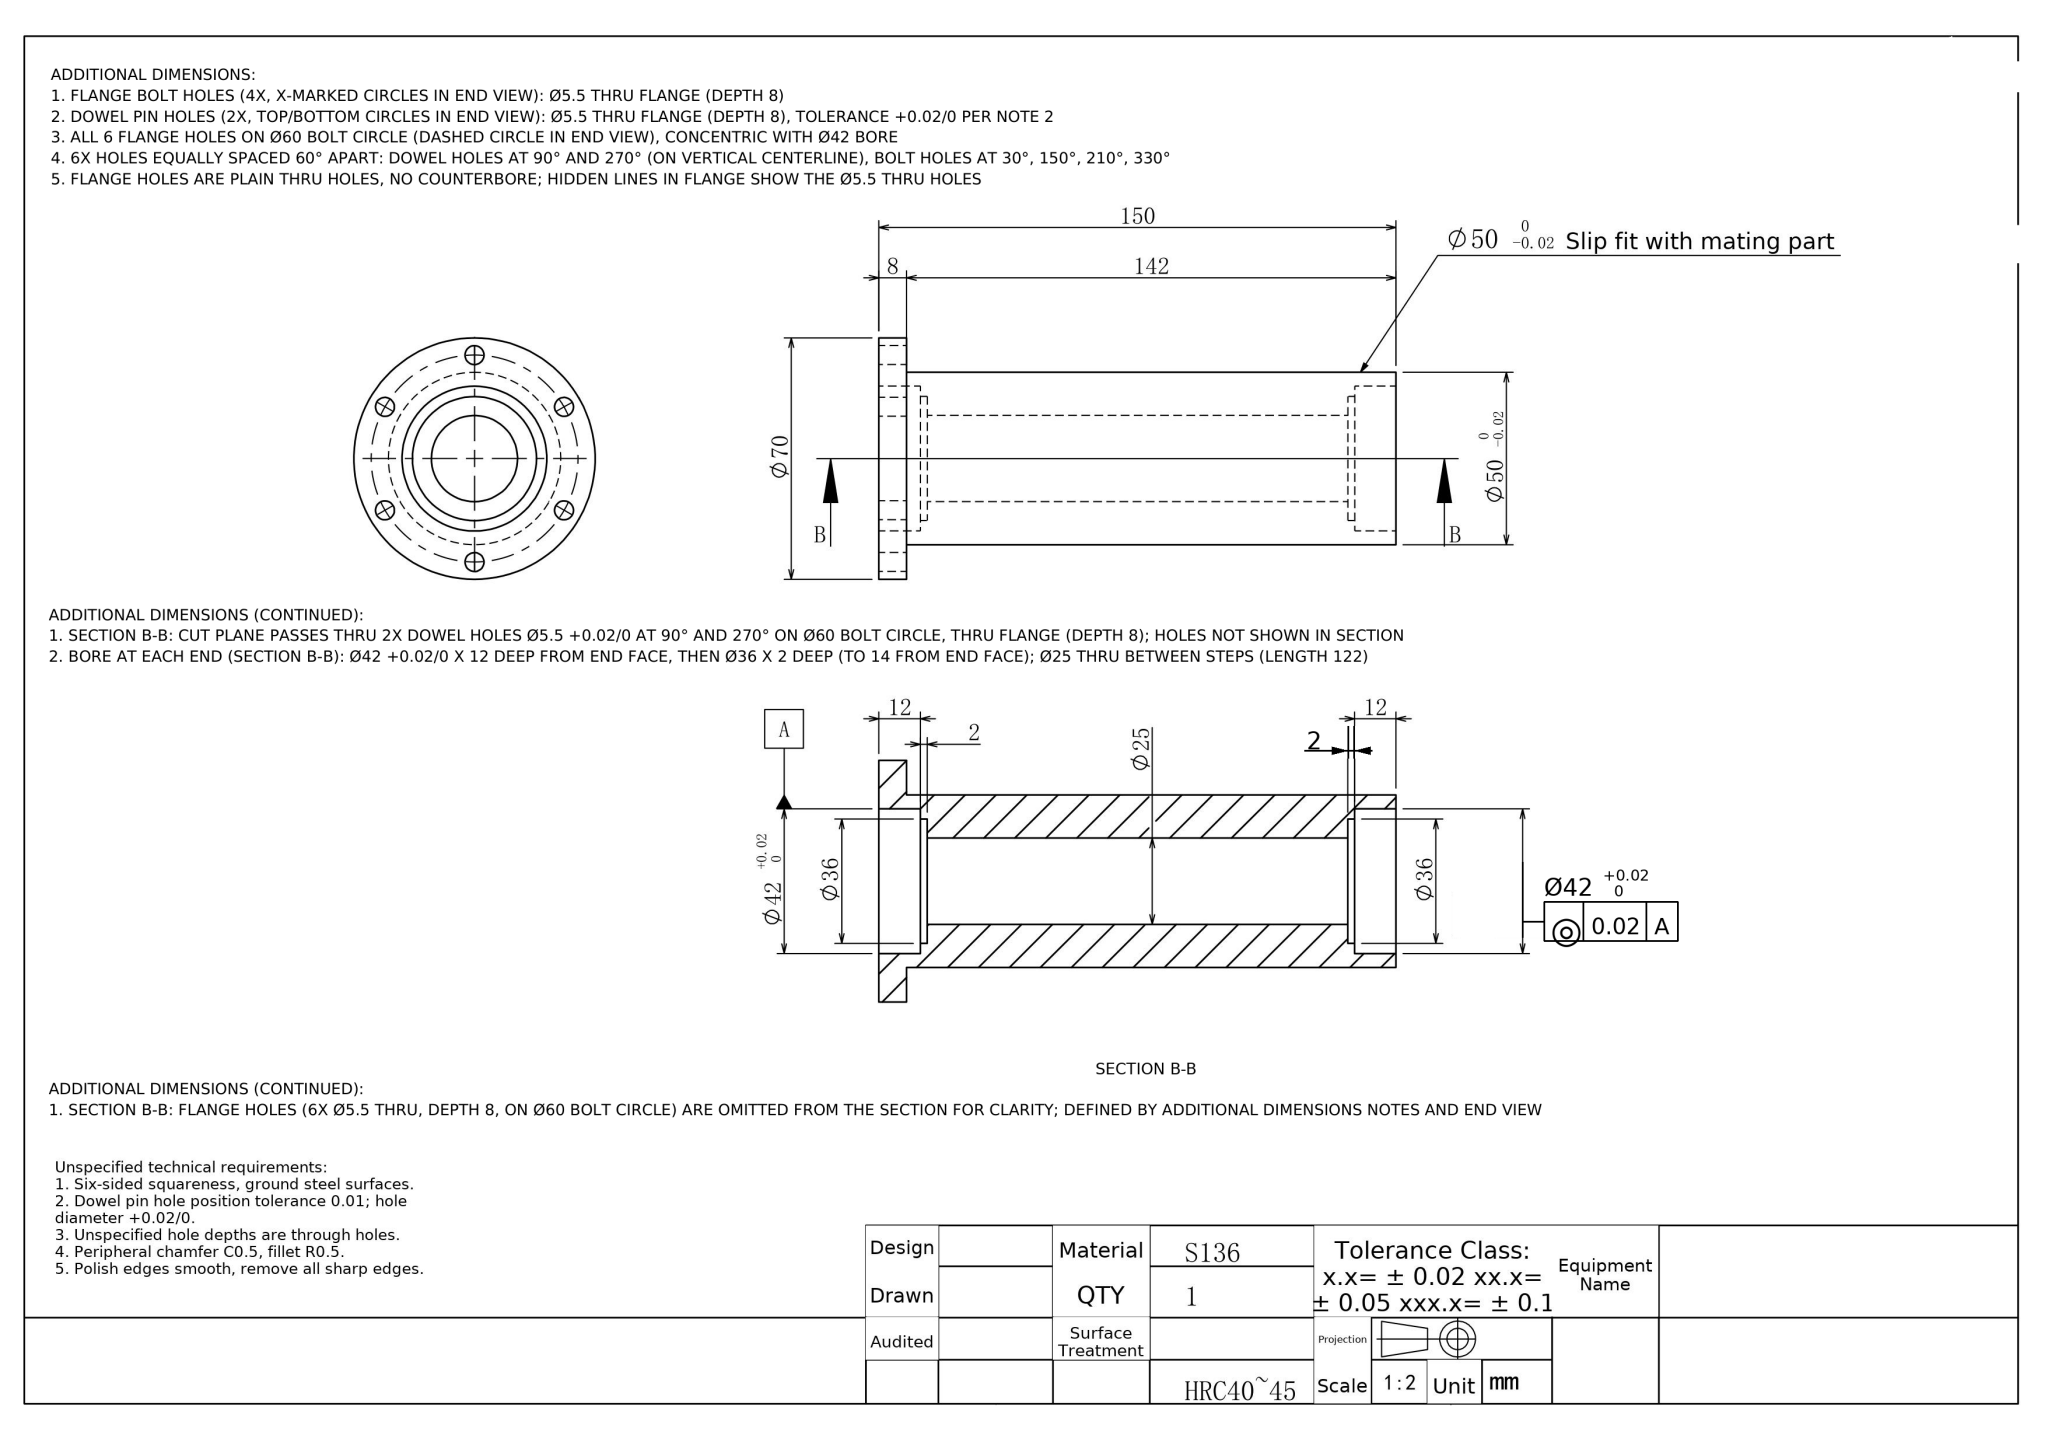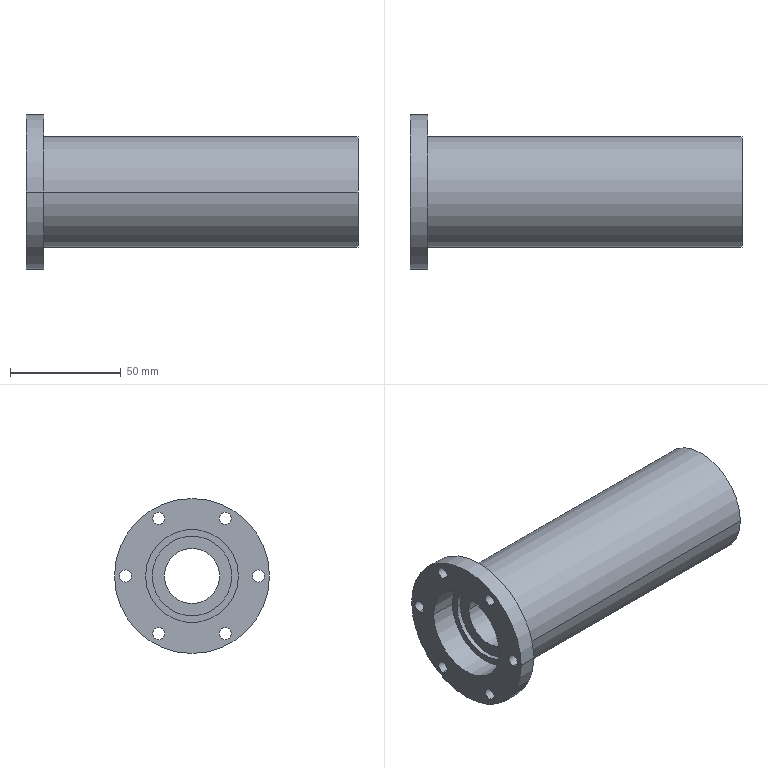Part | NX | mm | 1 solid | 33 faces | box 150 x 70 x 70 mm | volume 211255 mm3 | cylinder 26 | plane 7 | commonest cylinder face diameters 5.5 x12 36 x4 42 x4 50 x2 70 x2 25 x2
STEP:
#1=CARTESIAN_POINT('',(136.,-18.,0.));
#2=VERTEX_POINT('',#1);
#3=CARTESIAN_POINT('',(136.,18.,0.));
#4=VERTEX_POINT('',#3);
#5=CARTESIAN_POINT('',(136.,-0.,0.));
#6=DIRECTION('',(1.,-0.,0.));
#7=DIRECTION('',(0.,1.,0.));
#8=AXIS2_PLACEMENT_3D('',#5,#6,#7);
#9=CIRCLE('',#8,18.);
#10=EDGE_CURVE('',#2,#4,#9,.T.);
#11=ORIENTED_EDGE('',*,*,#10,.F.);
#12=CARTESIAN_POINT('',(138.,-18.,0.));
#13=VERTEX_POINT('',#12);
#14=CARTESIAN_POINT('',(136.,-18.,0.));
#15=DIRECTION('',(1.,-0.,0.));
#16=VECTOR('',#15,1000.);
#17=LINE('',#14,#16);
#18=EDGE_CURVE('',#2,#13,#17,.T.);
#19=ORIENTED_EDGE('',*,*,#18,.T.);
#20=CARTESIAN_POINT('',(138.,18.,0.));
#21=VERTEX_POINT('',#20);
#22=CARTESIAN_POINT('',(138.,-0.,0.));
#23=DIRECTION('',(1.,-0.,0.));
#24=DIRECTION('',(0.,1.,0.));
#25=AXIS2_PLACEMENT_3D('',#22,#23,#24);
#26=CIRCLE('',#25,18.);
#27=EDGE_CURVE('',#13,#21,#26,.T.);
#28=ORIENTED_EDGE('',*,*,#27,.T.);
#29=CARTESIAN_POINT('',(136.,18.,0.));
#30=DIRECTION('',(1.,-0.,0.));
#31=VECTOR('',#30,1000.);
#32=LINE('',#29,#31);
#33=EDGE_CURVE('',#4,#21,#32,.T.);
#34=ORIENTED_EDGE('',*,*,#33,.F.);
#35=EDGE_LOOP('',(#11,#19,#28,#34));
#36=FACE_OUTER_BOUND('',#35,.T.);
#37=CARTESIAN_POINT('',(136.,-0.,0.));
#38=DIRECTION('',(1.,-0.,0.));
#39=DIRECTION('',(0.,1.,0.));
#40=AXIS2_PLACEMENT_3D('',#37,#38,#39);
#41=CYLINDRICAL_SURFACE('',#40,18.);
#42=ADVANCED_FACE('',(#36),#41,.F.);
#43=CARTESIAN_POINT('',(14.,18.,0.));
#44=VERTEX_POINT('',#43);
#45=CARTESIAN_POINT('',(14.,-18.,0.));
#46=VERTEX_POINT('',#45);
#47=CARTESIAN_POINT('',(14.,-0.,0.));
#48=DIRECTION('',(-1.,0.,0.));
#49=DIRECTION('',(-0.,-1.,0.));
#50=AXIS2_PLACEMENT_3D('',#47,#48,#49);
#51=CIRCLE('',#50,18.);
#52=EDGE_CURVE('',#44,#46,#51,.T.);
#53=ORIENTED_EDGE('',*,*,#52,.F.);
#54=CARTESIAN_POINT('',(12.,18.,0.));
#55=VERTEX_POINT('',#54);
#56=CARTESIAN_POINT('',(14.,18.,0.));
#57=DIRECTION('',(-1.,0.,0.));
#58=VECTOR('',#57,1000.);
#59=LINE('',#56,#58);
#60=EDGE_CURVE('',#44,#55,#59,.T.);
#61=ORIENTED_EDGE('',*,*,#60,.T.);
#62=CARTESIAN_POINT('',(12.,-18.,0.));
#63=VERTEX_POINT('',#62);
#64=CARTESIAN_POINT('',(12.,-0.,0.));
#65=DIRECTION('',(-1.,0.,0.));
#66=DIRECTION('',(-0.,-1.,0.));
#67=AXIS2_PLACEMENT_3D('',#64,#65,#66);
#68=CIRCLE('',#67,18.);
#69=EDGE_CURVE('',#55,#63,#68,.T.);
#70=ORIENTED_EDGE('',*,*,#69,.T.);
#71=CARTESIAN_POINT('',(14.,-18.,0.));
#72=DIRECTION('',(-1.,0.,0.));
#73=VECTOR('',#72,1000.);
#74=LINE('',#71,#73);
#75=EDGE_CURVE('',#46,#63,#74,.T.);
#76=ORIENTED_EDGE('',*,*,#75,.F.);
#77=EDGE_LOOP('',(#53,#61,#70,#76));
#78=FACE_OUTER_BOUND('',#77,.T.);
#79=CARTESIAN_POINT('',(14.,-0.,0.));
#80=DIRECTION('',(-1.,0.,0.));
#81=DIRECTION('',(-0.,-1.,0.));
#82=AXIS2_PLACEMENT_3D('',#79,#80,#81);
#83=CYLINDRICAL_SURFACE('',#82,18.);
#84=ADVANCED_FACE('',(#78),#83,.F.);
#85=CARTESIAN_POINT('',(8.,15.,-23.231));
#86=VERTEX_POINT('',#85);
#87=CARTESIAN_POINT('',(8.,15.,-28.731));
#88=VERTEX_POINT('',#87);
#89=CARTESIAN_POINT('',(8.,15.,-25.981));
#90=DIRECTION('',(1.,-0.,0.));
#91=DIRECTION('',(0.,1.,0.));
#92=AXIS2_PLACEMENT_3D('',#89,#90,#91);
#93=CIRCLE('',#92,2.75);
#94=EDGE_CURVE('',#86,#88,#93,.T.);
#95=ORIENTED_EDGE('',*,*,#94,.T.);
#96=CARTESIAN_POINT('',(0.,15.,-28.731));
#97=VERTEX_POINT('',#96);
#98=CARTESIAN_POINT('',(0.,15.,-28.731));
#99=DIRECTION('',(-1.,0.,0.));
#100=VECTOR('',#99,1000.);
#101=LINE('',#98,#100);
#102=EDGE_CURVE('',#88,#97,#101,.T.);
#103=ORIENTED_EDGE('',*,*,#102,.T.);
#104=CARTESIAN_POINT('',(0.,15.,-23.231));
#105=VERTEX_POINT('',#104);
#106=CARTESIAN_POINT('',(0.,15.,-25.981));
#107=DIRECTION('',(-1.,0.,0.));
#108=DIRECTION('',(0.,0.,1.));
#109=AXIS2_PLACEMENT_3D('',#106,#107,#108);
#110=CIRCLE('',#109,2.75);
#111=EDGE_CURVE('',#97,#105,#110,.T.);
#112=ORIENTED_EDGE('',*,*,#111,.T.);
#113=CARTESIAN_POINT('',(0.,15.,-23.231));
#114=DIRECTION('',(-1.,0.,0.));
#115=VECTOR('',#114,1000.);
#116=LINE('',#113,#115);
#117=EDGE_CURVE('',#86,#105,#116,.T.);
#118=ORIENTED_EDGE('',*,*,#117,.F.);
#119=EDGE_LOOP('',(#95,#103,#112,#118));
#120=FACE_OUTER_BOUND('',#119,.T.);
#121=CARTESIAN_POINT('',(0.,15.,-25.981));
#122=DIRECTION('',(-1.,0.,0.));
#123=DIRECTION('',(0.,0.,1.));
#124=AXIS2_PLACEMENT_3D('',#121,#122,#123);
#125=CYLINDRICAL_SURFACE('',#124,2.75);
#126=ADVANCED_FACE('',(#120),#125,.F.);
#127=CARTESIAN_POINT('',(8.,-15.,-23.231));
#128=VERTEX_POINT('',#127);
#129=CARTESIAN_POINT('',(8.,-15.,-28.731));
#130=VERTEX_POINT('',#129);
#131=CARTESIAN_POINT('',(8.,-15.,-25.981));
#132=DIRECTION('',(1.,-0.,0.));
#133=DIRECTION('',(0.,1.,0.));
#134=AXIS2_PLACEMENT_3D('',#131,#132,#133);
#135=CIRCLE('',#134,2.75);
#136=EDGE_CURVE('',#128,#130,#135,.T.);
#137=ORIENTED_EDGE('',*,*,#136,.T.);
#138=CARTESIAN_POINT('',(-0.,-15.,-28.731));
#139=VERTEX_POINT('',#138);
#140=CARTESIAN_POINT('',(-0.,-15.,-28.731));
#141=DIRECTION('',(-1.,0.,0.));
#142=VECTOR('',#141,1000.);
#143=LINE('',#140,#142);
#144=EDGE_CURVE('',#130,#139,#143,.T.);
#145=ORIENTED_EDGE('',*,*,#144,.T.);
#146=CARTESIAN_POINT('',(-0.,-15.,-23.231));
#147=VERTEX_POINT('',#146);
#148=CARTESIAN_POINT('',(-0.,-15.,-25.981));
#149=DIRECTION('',(-1.,0.,0.));
#150=DIRECTION('',(0.,0.,1.));
#151=AXIS2_PLACEMENT_3D('',#148,#149,#150);
#152=CIRCLE('',#151,2.75);
#153=EDGE_CURVE('',#139,#147,#152,.T.);
#154=ORIENTED_EDGE('',*,*,#153,.T.);
#155=CARTESIAN_POINT('',(-0.,-15.,-23.231));
#156=DIRECTION('',(-1.,0.,0.));
#157=VECTOR('',#156,1000.);
#158=LINE('',#155,#157);
#159=EDGE_CURVE('',#128,#147,#158,.T.);
#160=ORIENTED_EDGE('',*,*,#159,.F.);
#161=EDGE_LOOP('',(#137,#145,#154,#160));
#162=FACE_OUTER_BOUND('',#161,.T.);
#163=CARTESIAN_POINT('',(-0.,-15.,-25.981));
#164=DIRECTION('',(-1.,0.,0.));
#165=DIRECTION('',(0.,0.,1.));
#166=AXIS2_PLACEMENT_3D('',#163,#164,#165);
#167=CYLINDRICAL_SURFACE('',#166,2.75);
#168=ADVANCED_FACE('',(#162),#167,.F.);
#169=CARTESIAN_POINT('',(8.,-30.,2.75));
#170=VERTEX_POINT('',#169);
#171=CARTESIAN_POINT('',(8.,-30.,-2.75));
#172=VERTEX_POINT('',#171);
#173=CARTESIAN_POINT('',(8.,-30.,0.));
#174=DIRECTION('',(1.,-0.,0.));
#175=DIRECTION('',(0.,1.,0.));
#176=AXIS2_PLACEMENT_3D('',#173,#174,#175);
#177=CIRCLE('',#176,2.75);
#178=EDGE_CURVE('',#170,#172,#177,.T.);
#179=ORIENTED_EDGE('',*,*,#178,.T.);
#180=CARTESIAN_POINT('',(-0.,-30.,-2.75));
#181=VERTEX_POINT('',#180);
#182=CARTESIAN_POINT('',(-0.,-30.,-2.75));
#183=DIRECTION('',(-1.,0.,0.));
#184=VECTOR('',#183,1000.);
#185=LINE('',#182,#184);
#186=EDGE_CURVE('',#172,#181,#185,.T.);
#187=ORIENTED_EDGE('',*,*,#186,.T.);
#188=CARTESIAN_POINT('',(-0.,-30.,2.75));
#189=VERTEX_POINT('',#188);
#190=CARTESIAN_POINT('',(-0.,-30.,0.));
#191=DIRECTION('',(-1.,0.,0.));
#192=DIRECTION('',(0.,0.,1.));
#193=AXIS2_PLACEMENT_3D('',#190,#191,#192);
#194=CIRCLE('',#193,2.75);
#195=EDGE_CURVE('',#181,#189,#194,.T.);
#196=ORIENTED_EDGE('',*,*,#195,.T.);
#197=CARTESIAN_POINT('',(-0.,-30.,2.75));
#198=DIRECTION('',(-1.,0.,0.));
#199=VECTOR('',#198,1000.);
#200=LINE('',#197,#199);
#201=EDGE_CURVE('',#170,#189,#200,.T.);
#202=ORIENTED_EDGE('',*,*,#201,.F.);
#203=EDGE_LOOP('',(#179,#187,#196,#202));
#204=FACE_OUTER_BOUND('',#203,.T.);
#205=CARTESIAN_POINT('',(-0.,-30.,0.));
#206=DIRECTION('',(-1.,0.,0.));
#207=DIRECTION('',(0.,0.,1.));
#208=AXIS2_PLACEMENT_3D('',#205,#206,#207);
#209=CYLINDRICAL_SURFACE('',#208,2.75);
#210=ADVANCED_FACE('',(#204),#209,.F.);
#211=CARTESIAN_POINT('',(8.,-15.,28.731));
#212=VERTEX_POINT('',#211);
#213=CARTESIAN_POINT('',(8.,-15.,23.231));
#214=VERTEX_POINT('',#213);
#215=CARTESIAN_POINT('',(8.,-15.,25.981));
#216=DIRECTION('',(1.,-0.,0.));
#217=DIRECTION('',(0.,1.,0.));
#218=AXIS2_PLACEMENT_3D('',#215,#216,#217);
#219=CIRCLE('',#218,2.75);
#220=EDGE_CURVE('',#212,#214,#219,.T.);
#221=ORIENTED_EDGE('',*,*,#220,.T.);
#222=CARTESIAN_POINT('',(-0.,-15.,23.231));
#223=VERTEX_POINT('',#222);
#224=CARTESIAN_POINT('',(-0.,-15.,23.231));
#225=DIRECTION('',(-1.,0.,0.));
#226=VECTOR('',#225,1000.);
#227=LINE('',#224,#226);
#228=EDGE_CURVE('',#214,#223,#227,.T.);
#229=ORIENTED_EDGE('',*,*,#228,.T.);
#230=CARTESIAN_POINT('',(-0.,-15.,28.731));
#231=VERTEX_POINT('',#230);
#232=CARTESIAN_POINT('',(-0.,-15.,25.981));
#233=DIRECTION('',(-1.,0.,0.));
#234=DIRECTION('',(0.,0.,1.));
#235=AXIS2_PLACEMENT_3D('',#232,#233,#234);
#236=CIRCLE('',#235,2.75);
#237=EDGE_CURVE('',#223,#231,#236,.T.);
#238=ORIENTED_EDGE('',*,*,#237,.T.);
#239=CARTESIAN_POINT('',(-0.,-15.,28.731));
#240=DIRECTION('',(-1.,0.,0.));
#241=VECTOR('',#240,1000.);
#242=LINE('',#239,#241);
#243=EDGE_CURVE('',#212,#231,#242,.T.);
#244=ORIENTED_EDGE('',*,*,#243,.F.);
#245=EDGE_LOOP('',(#221,#229,#238,#244));
#246=FACE_OUTER_BOUND('',#245,.T.);
#247=CARTESIAN_POINT('',(-0.,-15.,25.981));
#248=DIRECTION('',(-1.,0.,0.));
#249=DIRECTION('',(0.,0.,1.));
#250=AXIS2_PLACEMENT_3D('',#247,#248,#249);
#251=CYLINDRICAL_SURFACE('',#250,2.75);
#252=ADVANCED_FACE('',(#246),#251,.F.);
#253=CARTESIAN_POINT('',(8.,15.,28.731));
#254=VERTEX_POINT('',#253);
#255=CARTESIAN_POINT('',(8.,15.,23.231));
#256=VERTEX_POINT('',#255);
#257=CARTESIAN_POINT('',(8.,15.,25.981));
#258=DIRECTION('',(1.,-0.,0.));
#259=DIRECTION('',(0.,1.,0.));
#260=AXIS2_PLACEMENT_3D('',#257,#258,#259);
#261=CIRCLE('',#260,2.75);
#262=EDGE_CURVE('',#254,#256,#261,.T.);
#263=ORIENTED_EDGE('',*,*,#262,.T.);
#264=CARTESIAN_POINT('',(0.,15.,23.231));
#265=VERTEX_POINT('',#264);
#266=CARTESIAN_POINT('',(0.,15.,23.231));
#267=DIRECTION('',(-1.,0.,0.));
#268=VECTOR('',#267,1000.);
#269=LINE('',#266,#268);
#270=EDGE_CURVE('',#256,#265,#269,.T.);
#271=ORIENTED_EDGE('',*,*,#270,.T.);
#272=CARTESIAN_POINT('',(0.,15.,28.731));
#273=VERTEX_POINT('',#272);
#274=CARTESIAN_POINT('',(0.,15.,25.981));
#275=DIRECTION('',(-1.,0.,0.));
#276=DIRECTION('',(0.,0.,1.));
#277=AXIS2_PLACEMENT_3D('',#274,#275,#276);
#278=CIRCLE('',#277,2.75);
#279=EDGE_CURVE('',#265,#273,#278,.T.);
#280=ORIENTED_EDGE('',*,*,#279,.T.);
#281=CARTESIAN_POINT('',(0.,15.,28.731));
#282=DIRECTION('',(-1.,0.,0.));
#283=VECTOR('',#282,1000.);
#284=LINE('',#281,#283);
#285=EDGE_CURVE('',#254,#273,#284,.T.);
#286=ORIENTED_EDGE('',*,*,#285,.F.);
#287=EDGE_LOOP('',(#263,#271,#280,#286));
#288=FACE_OUTER_BOUND('',#287,.T.);
#289=CARTESIAN_POINT('',(0.,15.,25.981));
#290=DIRECTION('',(-1.,0.,0.));
#291=DIRECTION('',(0.,0.,1.));
#292=AXIS2_PLACEMENT_3D('',#289,#290,#291);
#293=CYLINDRICAL_SURFACE('',#292,2.75);
#294=ADVANCED_FACE('',(#288),#293,.F.);
#295=CARTESIAN_POINT('',(8.,30.,2.75));
#296=VERTEX_POINT('',#295);
#297=CARTESIAN_POINT('',(8.,30.,-2.75));
#298=VERTEX_POINT('',#297);
#299=CARTESIAN_POINT('',(8.,30.,0.));
#300=DIRECTION('',(1.,-0.,0.));
#301=DIRECTION('',(0.,1.,0.));
#302=AXIS2_PLACEMENT_3D('',#299,#300,#301);
#303=CIRCLE('',#302,2.75);
#304=EDGE_CURVE('',#296,#298,#303,.T.);
#305=ORIENTED_EDGE('',*,*,#304,.T.);
#306=CARTESIAN_POINT('',(0.,30.,-2.75));
#307=VERTEX_POINT('',#306);
#308=CARTESIAN_POINT('',(0.,30.,-2.75));
#309=DIRECTION('',(-1.,0.,0.));
#310=VECTOR('',#309,1000.);
#311=LINE('',#308,#310);
#312=EDGE_CURVE('',#298,#307,#311,.T.);
#313=ORIENTED_EDGE('',*,*,#312,.T.);
#314=CARTESIAN_POINT('',(0.,30.,2.75));
#315=VERTEX_POINT('',#314);
#316=CARTESIAN_POINT('',(0.,30.,0.));
#317=DIRECTION('',(-1.,0.,0.));
#318=DIRECTION('',(0.,0.,1.));
#319=AXIS2_PLACEMENT_3D('',#316,#317,#318);
#320=CIRCLE('',#319,2.75);
#321=EDGE_CURVE('',#307,#315,#320,.T.);
#322=ORIENTED_EDGE('',*,*,#321,.T.);
#323=CARTESIAN_POINT('',(0.,30.,2.75));
#324=DIRECTION('',(-1.,0.,0.));
#325=VECTOR('',#324,1000.);
#326=LINE('',#323,#325);
#327=EDGE_CURVE('',#296,#315,#326,.T.);
#328=ORIENTED_EDGE('',*,*,#327,.F.);
#329=EDGE_LOOP('',(#305,#313,#322,#328));
#330=FACE_OUTER_BOUND('',#329,.T.);
#331=CARTESIAN_POINT('',(0.,30.,0.));
#332=DIRECTION('',(-1.,0.,0.));
#333=DIRECTION('',(0.,0.,1.));
#334=AXIS2_PLACEMENT_3D('',#331,#332,#333);
#335=CYLINDRICAL_SURFACE('',#334,2.75);
#336=ADVANCED_FACE('',(#330),#335,.F.);
#337=CARTESIAN_POINT('',(12.,21.,0.));
#338=VERTEX_POINT('',#337);
#339=CARTESIAN_POINT('',(12.,-21.,0.));
#340=VERTEX_POINT('',#339);
#341=CARTESIAN_POINT('',(12.,-0.,0.));
#342=DIRECTION('',(-1.,0.,0.));
#343=DIRECTION('',(-0.,-1.,0.));
#344=AXIS2_PLACEMENT_3D('',#341,#342,#343);
#345=CIRCLE('',#344,21.);
#346=EDGE_CURVE('',#338,#340,#345,.T.);
#347=ORIENTED_EDGE('',*,*,#346,.F.);
#348=CARTESIAN_POINT('',(0.,21.,0.));
#349=VERTEX_POINT('',#348);
#350=CARTESIAN_POINT('',(12.,21.,0.));
#351=DIRECTION('',(-1.,0.,0.));
#352=VECTOR('',#351,1000.);
#353=LINE('',#350,#352);
#354=EDGE_CURVE('',#338,#349,#353,.T.);
#355=ORIENTED_EDGE('',*,*,#354,.T.);
#356=CARTESIAN_POINT('',(-0.,-21.,0.));
#357=VERTEX_POINT('',#356);
#358=CARTESIAN_POINT('',(0.,0.,0.));
#359=DIRECTION('',(-1.,0.,0.));
#360=DIRECTION('',(-0.,-1.,0.));
#361=AXIS2_PLACEMENT_3D('',#358,#359,#360);
#362=CIRCLE('',#361,21.);
#363=EDGE_CURVE('',#349,#357,#362,.T.);
#364=ORIENTED_EDGE('',*,*,#363,.T.);
#365=CARTESIAN_POINT('',(12.,-21.,0.));
#366=DIRECTION('',(-1.,0.,0.));
#367=VECTOR('',#366,1000.);
#368=LINE('',#365,#367);
#369=EDGE_CURVE('',#340,#357,#368,.T.);
#370=ORIENTED_EDGE('',*,*,#369,.F.);
#371=EDGE_LOOP('',(#347,#355,#364,#370));
#372=FACE_OUTER_BOUND('',#371,.T.);
#373=CARTESIAN_POINT('',(12.,-0.,0.));
#374=DIRECTION('',(-1.,0.,0.));
#375=DIRECTION('',(-0.,-1.,0.));
#376=AXIS2_PLACEMENT_3D('',#373,#374,#375);
#377=CYLINDRICAL_SURFACE('',#376,21.);
#378=ADVANCED_FACE('',(#372),#377,.F.);
#379=CARTESIAN_POINT('',(138.,-21.,0.));
#380=VERTEX_POINT('',#379);
#381=CARTESIAN_POINT('',(138.,21.,0.));
#382=VERTEX_POINT('',#381);
#383=CARTESIAN_POINT('',(138.,-0.,0.));
#384=DIRECTION('',(1.,-0.,0.));
#385=DIRECTION('',(0.,1.,0.));
#386=AXIS2_PLACEMENT_3D('',#383,#384,#385);
#387=CIRCLE('',#386,21.);
#388=EDGE_CURVE('',#380,#382,#387,.T.);
#389=ORIENTED_EDGE('',*,*,#388,.F.);
#390=CARTESIAN_POINT('',(150.,-21.,0.));
#391=VERTEX_POINT('',#390);
#392=CARTESIAN_POINT('',(138.,-21.,0.));
#393=DIRECTION('',(1.,-0.,0.));
#394=VECTOR('',#393,1000.);
#395=LINE('',#392,#394);
#396=EDGE_CURVE('',#380,#391,#395,.T.);
#397=ORIENTED_EDGE('',*,*,#396,.T.);
#398=CARTESIAN_POINT('',(150.,21.,0.));
#399=VERTEX_POINT('',#398);
#400=CARTESIAN_POINT('',(150.,-0.,0.));
#401=DIRECTION('',(1.,-0.,0.));
#402=DIRECTION('',(0.,1.,0.));
#403=AXIS2_PLACEMENT_3D('',#400,#401,#402);
#404=CIRCLE('',#403,21.);
#405=EDGE_CURVE('',#391,#399,#404,.T.);
#406=ORIENTED_EDGE('',*,*,#405,.T.);
#407=CARTESIAN_POINT('',(138.,21.,0.));
#408=DIRECTION('',(1.,-0.,0.));
#409=VECTOR('',#408,1000.);
#410=LINE('',#407,#409);
#411=EDGE_CURVE('',#382,#399,#410,.T.);
#412=ORIENTED_EDGE('',*,*,#411,.F.);
#413=EDGE_LOOP('',(#389,#397,#406,#412));
#414=FACE_OUTER_BOUND('',#413,.T.);
#415=CARTESIAN_POINT('',(138.,-0.,0.));
#416=DIRECTION('',(1.,-0.,0.));
#417=DIRECTION('',(0.,1.,0.));
#418=AXIS2_PLACEMENT_3D('',#415,#416,#417);
#419=CYLINDRICAL_SURFACE('',#418,21.);
#420=ADVANCED_FACE('',(#414),#419,.F.);
#421=CARTESIAN_POINT('',(8.,25.,0.));
#422=VERTEX_POINT('',#421);
#423=CARTESIAN_POINT('',(8.,-25.,0.));
#424=VERTEX_POINT('',#423);
#425=CARTESIAN_POINT('',(8.,-0.,0.));
#426=DIRECTION('',(1.,-0.,0.));
#427=DIRECTION('',(0.,1.,0.));
#428=AXIS2_PLACEMENT_3D('',#425,#426,#427);
#429=CIRCLE('',#428,25.);
#430=EDGE_CURVE('',#422,#424,#429,.T.);
#431=ORIENTED_EDGE('',*,*,#430,.T.);
#432=CARTESIAN_POINT('',(150.,-25.,0.));
#433=VERTEX_POINT('',#432);
#434=CARTESIAN_POINT('',(150.,-25.,0.));
#435=DIRECTION('',(1.,-0.,0.));
#436=VECTOR('',#435,1000.);
#437=LINE('',#434,#436);
#438=EDGE_CURVE('',#424,#433,#437,.T.);
#439=ORIENTED_EDGE('',*,*,#438,.T.);
#440=CARTESIAN_POINT('',(150.,25.,0.));
#441=VERTEX_POINT('',#440);
#442=CARTESIAN_POINT('',(150.,-0.,0.));
#443=DIRECTION('',(1.,-0.,0.));
#444=DIRECTION('',(0.,1.,0.));
#445=AXIS2_PLACEMENT_3D('',#442,#443,#444);
#446=CIRCLE('',#445,25.);
#447=EDGE_CURVE('',#441,#433,#446,.T.);
#448=ORIENTED_EDGE('',*,*,#447,.F.);
#449=CARTESIAN_POINT('',(150.,25.,0.));
#450=DIRECTION('',(1.,-0.,0.));
#451=VECTOR('',#450,1000.);
#452=LINE('',#449,#451);
#453=EDGE_CURVE('',#422,#441,#452,.T.);
#454=ORIENTED_EDGE('',*,*,#453,.F.);
#455=EDGE_LOOP('',(#431,#439,#448,#454));
#456=FACE_OUTER_BOUND('',#455,.T.);
#457=CARTESIAN_POINT('',(150.,-0.,0.));
#458=DIRECTION('',(1.,-0.,0.));
#459=DIRECTION('',(0.,1.,0.));
#460=AXIS2_PLACEMENT_3D('',#457,#458,#459);
#461=CYLINDRICAL_SURFACE('',#460,25.);
#462=ADVANCED_FACE('',(#456),#461,.T.);
#463=CARTESIAN_POINT('',(0.,35.,0.));
#464=VERTEX_POINT('',#463);
#465=CARTESIAN_POINT('',(-0.,-35.,0.));
#466=VERTEX_POINT('',#465);
#467=CARTESIAN_POINT('',(0.,0.,0.));
#468=DIRECTION('',(1.,-0.,0.));
#469=DIRECTION('',(0.,1.,0.));
#470=AXIS2_PLACEMENT_3D('',#467,#468,#469);
#471=CIRCLE('',#470,35.);
#472=EDGE_CURVE('',#464,#466,#471,.T.);
#473=ORIENTED_EDGE('',*,*,#472,.T.);
#474=CARTESIAN_POINT('',(8.,-35.,0.));
#475=VERTEX_POINT('',#474);
#476=CARTESIAN_POINT('',(150.,-35.,0.));
#477=DIRECTION('',(1.,-0.,0.));
#478=VECTOR('',#477,1000.);
#479=LINE('',#476,#478);
#480=EDGE_CURVE('',#466,#475,#479,.T.);
#481=ORIENTED_EDGE('',*,*,#480,.T.);
#482=CARTESIAN_POINT('',(8.,35.,0.));
#483=VERTEX_POINT('',#482);
#484=CARTESIAN_POINT('',(8.,-0.,0.));
#485=DIRECTION('',(1.,-0.,0.));
#486=DIRECTION('',(0.,1.,0.));
#487=AXIS2_PLACEMENT_3D('',#484,#485,#486);
#488=CIRCLE('',#487,35.);
#489=EDGE_CURVE('',#483,#475,#488,.T.);
#490=ORIENTED_EDGE('',*,*,#489,.F.);
#491=CARTESIAN_POINT('',(150.,35.,0.));
#492=DIRECTION('',(1.,-0.,0.));
#493=VECTOR('',#492,1000.);
#494=LINE('',#491,#493);
#495=EDGE_CURVE('',#464,#483,#494,.T.);
#496=ORIENTED_EDGE('',*,*,#495,.F.);
#497=EDGE_LOOP('',(#473,#481,#490,#496));
#498=FACE_OUTER_BOUND('',#497,.T.);
#499=CARTESIAN_POINT('',(150.,-0.,0.));
#500=DIRECTION('',(1.,-0.,0.));
#501=DIRECTION('',(0.,1.,0.));
#502=AXIS2_PLACEMENT_3D('',#499,#500,#501);
#503=CYLINDRICAL_SURFACE('',#502,35.);
#504=ADVANCED_FACE('',(#498),#503,.T.);
#505=CARTESIAN_POINT('',(136.,12.5,0.));
#506=VERTEX_POINT('',#505);
#507=CARTESIAN_POINT('',(136.,-12.5,0.));
#508=VERTEX_POINT('',#507);
#509=CARTESIAN_POINT('',(136.,-0.,0.));
#510=DIRECTION('',(-1.,0.,0.));
#511=DIRECTION('',(0.,1.,0.));
#512=AXIS2_PLACEMENT_3D('',#509,#510,#511);
#513=CIRCLE('',#512,12.5);
#514=EDGE_CURVE('',#506,#508,#513,.T.);
#515=ORIENTED_EDGE('',*,*,#514,.F.);
#516=CARTESIAN_POINT('',(14.,12.5,0.));
#517=VERTEX_POINT('',#516);
#518=CARTESIAN_POINT('',(150.,12.5,0.));
#519=DIRECTION('',(-1.,0.,0.));
#520=VECTOR('',#519,1000.);
#521=LINE('',#518,#520);
#522=EDGE_CURVE('',#506,#517,#521,.T.);
#523=ORIENTED_EDGE('',*,*,#522,.T.);
#524=CARTESIAN_POINT('',(14.,-12.5,0.));
#525=VERTEX_POINT('',#524);
#526=CARTESIAN_POINT('',(14.,-0.,0.));
#527=DIRECTION('',(1.,-0.,0.));
#528=DIRECTION('',(-0.,-1.,0.));
#529=AXIS2_PLACEMENT_3D('',#526,#527,#528);
#530=CIRCLE('',#529,12.5);
#531=EDGE_CURVE('',#525,#517,#530,.T.);
#532=ORIENTED_EDGE('',*,*,#531,.F.);
#533=CARTESIAN_POINT('',(150.,-12.5,0.));
#534=DIRECTION('',(-1.,0.,0.));
#535=VECTOR('',#534,1000.);
#536=LINE('',#533,#535);
#537=EDGE_CURVE('',#508,#525,#536,.T.);
#538=ORIENTED_EDGE('',*,*,#537,.F.);
#539=EDGE_LOOP('',(#515,#523,#532,#538));
#540=FACE_OUTER_BOUND('',#539,.T.);
#541=CARTESIAN_POINT('',(150.,-0.,0.));
#542=DIRECTION('',(-1.,0.,0.));
#543=DIRECTION('',(0.,-1.,0.));
#544=AXIS2_PLACEMENT_3D('',#541,#542,#543);
#545=CYLINDRICAL_SURFACE('',#544,12.5);
#546=ADVANCED_FACE('',(#540),#545,.F.);
#547=ORIENTED_EDGE('',*,*,#522,.F.);
#548=CARTESIAN_POINT('',(136.,-0.,0.));
#549=DIRECTION('',(-1.,0.,0.));
#550=DIRECTION('',(0.,1.,0.));
#551=AXIS2_PLACEMENT_3D('',#548,#549,#550);
#552=CIRCLE('',#551,12.5);
#553=EDGE_CURVE('',#508,#506,#552,.T.);
#554=ORIENTED_EDGE('',*,*,#553,.F.);
#555=ORIENTED_EDGE('',*,*,#537,.T.);
#556=CARTESIAN_POINT('',(14.,-0.,0.));
#557=DIRECTION('',(1.,-0.,0.));
#558=DIRECTION('',(-0.,-1.,0.));
#559=AXIS2_PLACEMENT_3D('',#556,#557,#558);
#560=CIRCLE('',#559,12.5);
#561=EDGE_CURVE('',#517,#525,#560,.T.);
#562=ORIENTED_EDGE('',*,*,#561,.F.);
#563=EDGE_LOOP('',(#547,#554,#555,#562));
#564=FACE_OUTER_BOUND('',#563,.T.);
#565=CARTESIAN_POINT('',(150.,-0.,0.));
#566=DIRECTION('',(-1.,0.,0.));
#567=DIRECTION('',(0.,-1.,0.));
#568=AXIS2_PLACEMENT_3D('',#565,#566,#567);
#569=CYLINDRICAL_SURFACE('',#568,12.5);
#570=ADVANCED_FACE('',(#564),#569,.F.);
#571=CARTESIAN_POINT('',(0.,15.,-25.981));
#572=DIRECTION('',(-1.,0.,0.));
#573=DIRECTION('',(0.,0.,1.));
#574=AXIS2_PLACEMENT_3D('',#571,#572,#573);
#575=CIRCLE('',#574,2.75);
#576=EDGE_CURVE('',#105,#97,#575,.T.);
#577=ORIENTED_EDGE('',*,*,#576,.F.);
#578=ORIENTED_EDGE('',*,*,#111,.F.);
#579=EDGE_LOOP('',(#577,#578));
#580=FACE_BOUND('',#579,.T.);
#581=CARTESIAN_POINT('',(-0.,-15.,-25.981));
#582=DIRECTION('',(-1.,0.,0.));
#583=DIRECTION('',(0.,0.,1.));
#584=AXIS2_PLACEMENT_3D('',#581,#582,#583);
#585=CIRCLE('',#584,2.75);
#586=EDGE_CURVE('',#147,#139,#585,.T.);
#587=ORIENTED_EDGE('',*,*,#586,.F.);
#588=ORIENTED_EDGE('',*,*,#153,.F.);
#589=EDGE_LOOP('',(#587,#588));
#590=FACE_BOUND('',#589,.T.);
#591=CARTESIAN_POINT('',(-0.,-30.,0.));
#592=DIRECTION('',(-1.,0.,0.));
#593=DIRECTION('',(0.,0.,1.));
#594=AXIS2_PLACEMENT_3D('',#591,#592,#593);
#595=CIRCLE('',#594,2.75);
#596=EDGE_CURVE('',#189,#181,#595,.T.);
#597=ORIENTED_EDGE('',*,*,#596,.F.);
#598=ORIENTED_EDGE('',*,*,#195,.F.);
#599=EDGE_LOOP('',(#597,#598));
#600=FACE_BOUND('',#599,.T.);
#601=CARTESIAN_POINT('',(-0.,-15.,25.981));
#602=DIRECTION('',(-1.,0.,0.));
#603=DIRECTION('',(0.,0.,1.));
#604=AXIS2_PLACEMENT_3D('',#601,#602,#603);
#605=CIRCLE('',#604,2.75);
#606=EDGE_CURVE('',#231,#223,#605,.T.);
#607=ORIENTED_EDGE('',*,*,#606,.F.);
#608=ORIENTED_EDGE('',*,*,#237,.F.);
#609=EDGE_LOOP('',(#607,#608));
#610=FACE_BOUND('',#609,.T.);
#611=CARTESIAN_POINT('',(0.,15.,25.981));
#612=DIRECTION('',(-1.,0.,0.));
#613=DIRECTION('',(0.,0.,1.));
#614=AXIS2_PLACEMENT_3D('',#611,#612,#613);
#615=CIRCLE('',#614,2.75);
#616=EDGE_CURVE('',#273,#265,#615,.T.);
#617=ORIENTED_EDGE('',*,*,#616,.F.);
#618=ORIENTED_EDGE('',*,*,#279,.F.);
#619=EDGE_LOOP('',(#617,#618));
#620=FACE_BOUND('',#619,.T.);
#621=CARTESIAN_POINT('',(0.,30.,0.));
#622=DIRECTION('',(-1.,0.,0.));
#623=DIRECTION('',(0.,0.,1.));
#624=AXIS2_PLACEMENT_3D('',#621,#622,#623);
#625=CIRCLE('',#624,2.75);
#626=EDGE_CURVE('',#315,#307,#625,.T.);
#627=ORIENTED_EDGE('',*,*,#626,.F.);
#628=ORIENTED_EDGE('',*,*,#321,.F.);
#629=EDGE_LOOP('',(#627,#628));
#630=FACE_BOUND('',#629,.T.);
#631=CARTESIAN_POINT('',(0.,0.,0.));
#632=DIRECTION('',(-1.,0.,0.));
#633=DIRECTION('',(-0.,-1.,0.));
#634=AXIS2_PLACEMENT_3D('',#631,#632,#633);
#635=CIRCLE('',#634,21.);
#636=EDGE_CURVE('',#357,#349,#635,.T.);
#637=ORIENTED_EDGE('',*,*,#636,.F.);
#638=ORIENTED_EDGE('',*,*,#363,.F.);
#639=EDGE_LOOP('',(#637,#638));
#640=FACE_BOUND('',#639,.T.);
#641=ORIENTED_EDGE('',*,*,#472,.F.);
#642=CARTESIAN_POINT('',(0.,0.,0.));
#643=DIRECTION('',(1.,-0.,0.));
#644=DIRECTION('',(0.,1.,0.));
#645=AXIS2_PLACEMENT_3D('',#642,#643,#644);
#646=CIRCLE('',#645,35.);
#647=EDGE_CURVE('',#466,#464,#646,.T.);
#648=ORIENTED_EDGE('',*,*,#647,.F.);
#649=EDGE_LOOP('',(#641,#648));
#650=FACE_OUTER_BOUND('',#649,.T.);
#651=CARTESIAN_POINT('',(-0.,0.,0.));
#652=DIRECTION('',(-1.,0.,0.));
#653=DIRECTION('',(-0.,-1.,0.));
#654=AXIS2_PLACEMENT_3D('',#651,#652,#653);
#655=PLANE('',#654);
#656=ADVANCED_FACE('',(#580,#590,#600,#610,#620,#630,#640,#650),#655,.T.);
#657=ORIENTED_EDGE('',*,*,#480,.F.);
#658=ORIENTED_EDGE('',*,*,#647,.T.);
#659=ORIENTED_EDGE('',*,*,#495,.T.);
#660=CARTESIAN_POINT('',(8.,-0.,0.));
#661=DIRECTION('',(1.,-0.,0.));
#662=DIRECTION('',(0.,1.,0.));
#663=AXIS2_PLACEMENT_3D('',#660,#661,#662);
#664=CIRCLE('',#663,35.);
#665=EDGE_CURVE('',#475,#483,#664,.T.);
#666=ORIENTED_EDGE('',*,*,#665,.F.);
#667=EDGE_LOOP('',(#657,#658,#659,#666));
#668=FACE_OUTER_BOUND('',#667,.T.);
#669=CARTESIAN_POINT('',(150.,-0.,0.));
#670=DIRECTION('',(1.,-0.,0.));
#671=DIRECTION('',(0.,1.,0.));
#672=AXIS2_PLACEMENT_3D('',#669,#670,#671);
#673=CYLINDRICAL_SURFACE('',#672,35.);
#674=ADVANCED_FACE('',(#668),#673,.T.);
#675=ORIENTED_EDGE('',*,*,#94,.F.);
#676=CARTESIAN_POINT('',(8.,15.,-25.981));
#677=DIRECTION('',(1.,-0.,0.));
#678=DIRECTION('',(0.,1.,0.));
#679=AXIS2_PLACEMENT_3D('',#676,#677,#678);
#680=CIRCLE('',#679,2.75);
#681=EDGE_CURVE('',#88,#86,#680,.T.);
#682=ORIENTED_EDGE('',*,*,#681,.F.);
#683=EDGE_LOOP('',(#675,#682));
#684=FACE_BOUND('',#683,.T.);
#685=ORIENTED_EDGE('',*,*,#136,.F.);
#686=CARTESIAN_POINT('',(8.,-15.,-25.981));
#687=DIRECTION('',(1.,-0.,0.));
#688=DIRECTION('',(0.,1.,0.));
#689=AXIS2_PLACEMENT_3D('',#686,#687,#688);
#690=CIRCLE('',#689,2.75);
#691=EDGE_CURVE('',#130,#128,#690,.T.);
#692=ORIENTED_EDGE('',*,*,#691,.F.);
#693=EDGE_LOOP('',(#685,#692));
#694=FACE_BOUND('',#693,.T.);
#695=ORIENTED_EDGE('',*,*,#178,.F.);
#696=CARTESIAN_POINT('',(8.,-30.,0.));
#697=DIRECTION('',(1.,-0.,0.));
#698=DIRECTION('',(0.,1.,0.));
#699=AXIS2_PLACEMENT_3D('',#696,#697,#698);
#700=CIRCLE('',#699,2.75);
#701=EDGE_CURVE('',#172,#170,#700,.T.);
#702=ORIENTED_EDGE('',*,*,#701,.F.);
#703=EDGE_LOOP('',(#695,#702));
#704=FACE_BOUND('',#703,.T.);
#705=ORIENTED_EDGE('',*,*,#220,.F.);
#706=CARTESIAN_POINT('',(8.,-15.,25.981));
#707=DIRECTION('',(1.,-0.,0.));
#708=DIRECTION('',(0.,1.,0.));
#709=AXIS2_PLACEMENT_3D('',#706,#707,#708);
#710=CIRCLE('',#709,2.75);
#711=EDGE_CURVE('',#214,#212,#710,.T.);
#712=ORIENTED_EDGE('',*,*,#711,.F.);
#713=EDGE_LOOP('',(#705,#712));
#714=FACE_BOUND('',#713,.T.);
#715=ORIENTED_EDGE('',*,*,#262,.F.);
#716=CARTESIAN_POINT('',(8.,15.,25.981));
#717=DIRECTION('',(1.,-0.,0.));
#718=DIRECTION('',(0.,1.,0.));
#719=AXIS2_PLACEMENT_3D('',#716,#717,#718);
#720=CIRCLE('',#719,2.75);
#721=EDGE_CURVE('',#256,#254,#720,.T.);
#722=ORIENTED_EDGE('',*,*,#721,.F.);
#723=EDGE_LOOP('',(#715,#722));
#724=FACE_BOUND('',#723,.T.);
#725=ORIENTED_EDGE('',*,*,#304,.F.);
#726=CARTESIAN_POINT('',(8.,30.,0.));
#727=DIRECTION('',(1.,-0.,0.));
#728=DIRECTION('',(0.,1.,0.));
#729=AXIS2_PLACEMENT_3D('',#726,#727,#728);
#730=CIRCLE('',#729,2.75);
#731=EDGE_CURVE('',#298,#296,#730,.T.);
#732=ORIENTED_EDGE('',*,*,#731,.F.);
#733=EDGE_LOOP('',(#725,#732));
#734=FACE_BOUND('',#733,.T.);
#735=ORIENTED_EDGE('',*,*,#489,.T.);
#736=ORIENTED_EDGE('',*,*,#665,.T.);
#737=EDGE_LOOP('',(#735,#736));
#738=FACE_OUTER_BOUND('',#737,.T.);
#739=ORIENTED_EDGE('',*,*,#430,.F.);
#740=CARTESIAN_POINT('',(8.,-0.,0.));
#741=DIRECTION('',(1.,-0.,0.));
#742=DIRECTION('',(0.,1.,0.));
#743=AXIS2_PLACEMENT_3D('',#740,#741,#742);
#744=CIRCLE('',#743,25.);
#745=EDGE_CURVE('',#424,#422,#744,.T.);
#746=ORIENTED_EDGE('',*,*,#745,.F.);
#747=EDGE_LOOP('',(#739,#746));
#748=FACE_BOUND('',#747,.T.);
#749=CARTESIAN_POINT('',(8.,35.,0.));
#750=DIRECTION('',(1.,-0.,0.));
#751=DIRECTION('',(0.,1.,0.));
#752=AXIS2_PLACEMENT_3D('',#749,#750,#751);
#753=PLANE('',#752);
#754=ADVANCED_FACE('',(#684,#694,#704,#714,#724,#734,#738,#748),#753,.T.);
#755=ORIENTED_EDGE('',*,*,#438,.F.);
#756=ORIENTED_EDGE('',*,*,#745,.T.);
#757=ORIENTED_EDGE('',*,*,#453,.T.);
#758=CARTESIAN_POINT('',(150.,-0.,0.));
#759=DIRECTION('',(1.,-0.,0.));
#760=DIRECTION('',(0.,1.,0.));
#761=AXIS2_PLACEMENT_3D('',#758,#759,#760);
#762=CIRCLE('',#761,25.);
#763=EDGE_CURVE('',#433,#441,#762,.T.);
#764=ORIENTED_EDGE('',*,*,#763,.F.);
#765=EDGE_LOOP('',(#755,#756,#757,#764));
#766=FACE_OUTER_BOUND('',#765,.T.);
#767=CARTESIAN_POINT('',(150.,-0.,0.));
#768=DIRECTION('',(1.,-0.,0.));
#769=DIRECTION('',(0.,1.,0.));
#770=AXIS2_PLACEMENT_3D('',#767,#768,#769);
#771=CYLINDRICAL_SURFACE('',#770,25.);
#772=ADVANCED_FACE('',(#766),#771,.T.);
#773=CARTESIAN_POINT('',(150.,-0.,0.));
#774=DIRECTION('',(1.,-0.,0.));
#775=DIRECTION('',(0.,1.,0.));
#776=AXIS2_PLACEMENT_3D('',#773,#774,#775);
#777=CIRCLE('',#776,21.);
#778=EDGE_CURVE('',#399,#391,#777,.T.);
#779=ORIENTED_EDGE('',*,*,#778,.F.);
#780=ORIENTED_EDGE('',*,*,#405,.F.);
#781=EDGE_LOOP('',(#779,#780));
#782=FACE_BOUND('',#781,.T.);
#783=ORIENTED_EDGE('',*,*,#447,.T.);
#784=ORIENTED_EDGE('',*,*,#763,.T.);
#785=EDGE_LOOP('',(#783,#784));
#786=FACE_OUTER_BOUND('',#785,.T.);
#787=CARTESIAN_POINT('',(150.,25.,0.));
#788=DIRECTION('',(1.,-0.,0.));
#789=DIRECTION('',(0.,1.,0.));
#790=AXIS2_PLACEMENT_3D('',#787,#788,#789);
#791=PLANE('',#790);
#792=ADVANCED_FACE('',(#782,#786),#791,.T.);
#793=CARTESIAN_POINT('',(138.,-0.,0.));
#794=DIRECTION('',(1.,-0.,0.));
#795=DIRECTION('',(0.,1.,0.));
#796=AXIS2_PLACEMENT_3D('',#793,#794,#795);
#797=CIRCLE('',#796,18.);
#798=EDGE_CURVE('',#21,#13,#797,.T.);
#799=ORIENTED_EDGE('',*,*,#798,.F.);
#800=ORIENTED_EDGE('',*,*,#27,.F.);
#801=EDGE_LOOP('',(#799,#800));
#802=FACE_BOUND('',#801,.T.);
#803=CARTESIAN_POINT('',(138.,-0.,0.));
#804=DIRECTION('',(1.,-0.,0.));
#805=DIRECTION('',(0.,1.,0.));
#806=AXIS2_PLACEMENT_3D('',#803,#804,#805);
#807=CIRCLE('',#806,21.);
#808=EDGE_CURVE('',#382,#380,#807,.T.);
#809=ORIENTED_EDGE('',*,*,#808,.T.);
#810=ORIENTED_EDGE('',*,*,#388,.T.);
#811=EDGE_LOOP('',(#809,#810));
#812=FACE_OUTER_BOUND('',#811,.T.);
#813=CARTESIAN_POINT('',(138.,-0.,0.));
#814=DIRECTION('',(1.,-0.,0.));
#815=DIRECTION('',(0.,1.,0.));
#816=AXIS2_PLACEMENT_3D('',#813,#814,#815);
#817=PLANE('',#816);
#818=ADVANCED_FACE('',(#802,#812),#817,.T.);
#819=ORIENTED_EDGE('',*,*,#396,.F.);
#820=ORIENTED_EDGE('',*,*,#808,.F.);
#821=ORIENTED_EDGE('',*,*,#411,.T.);
#822=ORIENTED_EDGE('',*,*,#778,.T.);
#823=EDGE_LOOP('',(#819,#820,#821,#822));
#824=FACE_OUTER_BOUND('',#823,.T.);
#825=CARTESIAN_POINT('',(138.,-0.,0.));
#826=DIRECTION('',(1.,-0.,0.));
#827=DIRECTION('',(0.,1.,0.));
#828=AXIS2_PLACEMENT_3D('',#825,#826,#827);
#829=CYLINDRICAL_SURFACE('',#828,21.);
#830=ADVANCED_FACE('',(#824),#829,.F.);
#831=CARTESIAN_POINT('',(12.,-0.,0.));
#832=DIRECTION('',(-1.,0.,0.));
#833=DIRECTION('',(-0.,-1.,0.));
#834=AXIS2_PLACEMENT_3D('',#831,#832,#833);
#835=CIRCLE('',#834,18.);
#836=EDGE_CURVE('',#63,#55,#835,.T.);
#837=ORIENTED_EDGE('',*,*,#836,.F.);
#838=ORIENTED_EDGE('',*,*,#69,.F.);
#839=EDGE_LOOP('',(#837,#838));
#840=FACE_BOUND('',#839,.T.);
#841=CARTESIAN_POINT('',(12.,-0.,0.));
#842=DIRECTION('',(-1.,0.,0.));
#843=DIRECTION('',(-0.,-1.,0.));
#844=AXIS2_PLACEMENT_3D('',#841,#842,#843);
#845=CIRCLE('',#844,21.);
#846=EDGE_CURVE('',#340,#338,#845,.T.);
#847=ORIENTED_EDGE('',*,*,#846,.T.);
#848=ORIENTED_EDGE('',*,*,#346,.T.);
#849=EDGE_LOOP('',(#847,#848));
#850=FACE_OUTER_BOUND('',#849,.T.);
#851=CARTESIAN_POINT('',(12.,-0.,0.));
#852=DIRECTION('',(-1.,0.,0.));
#853=DIRECTION('',(-0.,-1.,0.));
#854=AXIS2_PLACEMENT_3D('',#851,#852,#853);
#855=PLANE('',#854);
#856=ADVANCED_FACE('',(#840,#850),#855,.T.);
#857=ORIENTED_EDGE('',*,*,#354,.F.);
#858=ORIENTED_EDGE('',*,*,#846,.F.);
#859=ORIENTED_EDGE('',*,*,#369,.T.);
#860=ORIENTED_EDGE('',*,*,#636,.T.);
#861=EDGE_LOOP('',(#857,#858,#859,#860));
#862=FACE_OUTER_BOUND('',#861,.T.);
#863=CARTESIAN_POINT('',(12.,-0.,0.));
#864=DIRECTION('',(-1.,0.,0.));
#865=DIRECTION('',(-0.,-1.,0.));
#866=AXIS2_PLACEMENT_3D('',#863,#864,#865);
#867=CYLINDRICAL_SURFACE('',#866,21.);
#868=ADVANCED_FACE('',(#862),#867,.F.);
#869=ORIENTED_EDGE('',*,*,#312,.F.);
#870=ORIENTED_EDGE('',*,*,#731,.T.);
#871=ORIENTED_EDGE('',*,*,#327,.T.);
#872=ORIENTED_EDGE('',*,*,#626,.T.);
#873=EDGE_LOOP('',(#869,#870,#871,#872));
#874=FACE_OUTER_BOUND('',#873,.T.);
#875=CARTESIAN_POINT('',(0.,30.,0.));
#876=DIRECTION('',(-1.,0.,0.));
#877=DIRECTION('',(0.,0.,1.));
#878=AXIS2_PLACEMENT_3D('',#875,#876,#877);
#879=CYLINDRICAL_SURFACE('',#878,2.75);
#880=ADVANCED_FACE('',(#874),#879,.F.);
#881=ORIENTED_EDGE('',*,*,#270,.F.);
#882=ORIENTED_EDGE('',*,*,#721,.T.);
#883=ORIENTED_EDGE('',*,*,#285,.T.);
#884=ORIENTED_EDGE('',*,*,#616,.T.);
#885=EDGE_LOOP('',(#881,#882,#883,#884));
#886=FACE_OUTER_BOUND('',#885,.T.);
#887=CARTESIAN_POINT('',(0.,15.,25.981));
#888=DIRECTION('',(-1.,0.,0.));
#889=DIRECTION('',(0.,0.,1.));
#890=AXIS2_PLACEMENT_3D('',#887,#888,#889);
#891=CYLINDRICAL_SURFACE('',#890,2.75);
#892=ADVANCED_FACE('',(#886),#891,.F.);
#893=ORIENTED_EDGE('',*,*,#228,.F.);
#894=ORIENTED_EDGE('',*,*,#711,.T.);
#895=ORIENTED_EDGE('',*,*,#243,.T.);
#896=ORIENTED_EDGE('',*,*,#606,.T.);
#897=EDGE_LOOP('',(#893,#894,#895,#896));
#898=FACE_OUTER_BOUND('',#897,.T.);
#899=CARTESIAN_POINT('',(-0.,-15.,25.981));
#900=DIRECTION('',(-1.,0.,0.));
#901=DIRECTION('',(0.,0.,1.));
#902=AXIS2_PLACEMENT_3D('',#899,#900,#901);
#903=CYLINDRICAL_SURFACE('',#902,2.75);
#904=ADVANCED_FACE('',(#898),#903,.F.);
#905=ORIENTED_EDGE('',*,*,#186,.F.);
#906=ORIENTED_EDGE('',*,*,#701,.T.);
#907=ORIENTED_EDGE('',*,*,#201,.T.);
#908=ORIENTED_EDGE('',*,*,#596,.T.);
#909=EDGE_LOOP('',(#905,#906,#907,#908));
#910=FACE_OUTER_BOUND('',#909,.T.);
#911=CARTESIAN_POINT('',(-0.,-30.,0.));
#912=DIRECTION('',(-1.,0.,0.));
#913=DIRECTION('',(0.,0.,1.));
#914=AXIS2_PLACEMENT_3D('',#911,#912,#913);
#915=CYLINDRICAL_SURFACE('',#914,2.75);
#916=ADVANCED_FACE('',(#910),#915,.F.);
#917=ORIENTED_EDGE('',*,*,#144,.F.);
#918=ORIENTED_EDGE('',*,*,#691,.T.);
#919=ORIENTED_EDGE('',*,*,#159,.T.);
#920=ORIENTED_EDGE('',*,*,#586,.T.);
#921=EDGE_LOOP('',(#917,#918,#919,#920));
#922=FACE_OUTER_BOUND('',#921,.T.);
#923=CARTESIAN_POINT('',(-0.,-15.,-25.981));
#924=DIRECTION('',(-1.,0.,0.));
#925=DIRECTION('',(0.,0.,1.));
#926=AXIS2_PLACEMENT_3D('',#923,#924,#925);
#927=CYLINDRICAL_SURFACE('',#926,2.75);
#928=ADVANCED_FACE('',(#922),#927,.F.);
#929=ORIENTED_EDGE('',*,*,#102,.F.);
#930=ORIENTED_EDGE('',*,*,#681,.T.);
#931=ORIENTED_EDGE('',*,*,#117,.T.);
#932=ORIENTED_EDGE('',*,*,#576,.T.);
#933=EDGE_LOOP('',(#929,#930,#931,#932));
#934=FACE_OUTER_BOUND('',#933,.T.);
#935=CARTESIAN_POINT('',(0.,15.,-25.981));
#936=DIRECTION('',(-1.,0.,0.));
#937=DIRECTION('',(0.,0.,1.));
#938=AXIS2_PLACEMENT_3D('',#935,#936,#937);
#939=CYLINDRICAL_SURFACE('',#938,2.75);
#940=ADVANCED_FACE('',(#934),#939,.F.);
#941=CARTESIAN_POINT('',(14.,-0.,0.));
#942=DIRECTION('',(-1.,0.,0.));
#943=DIRECTION('',(-0.,-1.,0.));
#944=AXIS2_PLACEMENT_3D('',#941,#942,#943);
#945=CIRCLE('',#944,18.);
#946=EDGE_CURVE('',#46,#44,#945,.T.);
#947=ORIENTED_EDGE('',*,*,#946,.T.);
#948=ORIENTED_EDGE('',*,*,#52,.T.);
#949=EDGE_LOOP('',(#947,#948));
#950=FACE_OUTER_BOUND('',#949,.T.);
#951=ORIENTED_EDGE('',*,*,#531,.T.);
#952=ORIENTED_EDGE('',*,*,#561,.T.);
#953=EDGE_LOOP('',(#951,#952));
#954=FACE_BOUND('',#953,.T.);
#955=CARTESIAN_POINT('',(14.,-0.,0.));
#956=DIRECTION('',(-1.,0.,0.));
#957=DIRECTION('',(-0.,-1.,0.));
#958=AXIS2_PLACEMENT_3D('',#955,#956,#957);
#959=PLANE('',#958);
#960=ADVANCED_FACE('',(#950,#954),#959,.T.);
#961=ORIENTED_EDGE('',*,*,#60,.F.);
#962=ORIENTED_EDGE('',*,*,#946,.F.);
#963=ORIENTED_EDGE('',*,*,#75,.T.);
#964=ORIENTED_EDGE('',*,*,#836,.T.);
#965=EDGE_LOOP('',(#961,#962,#963,#964));
#966=FACE_OUTER_BOUND('',#965,.T.);
#967=CARTESIAN_POINT('',(14.,-0.,0.));
#968=DIRECTION('',(-1.,0.,0.));
#969=DIRECTION('',(-0.,-1.,0.));
#970=AXIS2_PLACEMENT_3D('',#967,#968,#969);
#971=CYLINDRICAL_SURFACE('',#970,18.);
#972=ADVANCED_FACE('',(#966),#971,.F.);
#973=CARTESIAN_POINT('',(136.,-0.,0.));
#974=DIRECTION('',(1.,-0.,0.));
#975=DIRECTION('',(0.,1.,0.));
#976=AXIS2_PLACEMENT_3D('',#973,#974,#975);
#977=CIRCLE('',#976,18.);
#978=EDGE_CURVE('',#4,#2,#977,.T.);
#979=ORIENTED_EDGE('',*,*,#978,.T.);
#980=ORIENTED_EDGE('',*,*,#10,.T.);
#981=EDGE_LOOP('',(#979,#980));
#982=FACE_OUTER_BOUND('',#981,.T.);
#983=ORIENTED_EDGE('',*,*,#553,.T.);
#984=ORIENTED_EDGE('',*,*,#514,.T.);
#985=EDGE_LOOP('',(#983,#984));
#986=FACE_BOUND('',#985,.T.);
#987=CARTESIAN_POINT('',(136.,-0.,0.));
#988=DIRECTION('',(1.,-0.,0.));
#989=DIRECTION('',(0.,1.,0.));
#990=AXIS2_PLACEMENT_3D('',#987,#988,#989);
#991=PLANE('',#990);
#992=ADVANCED_FACE('',(#982,#986),#991,.T.);
#993=ORIENTED_EDGE('',*,*,#18,.F.);
#994=ORIENTED_EDGE('',*,*,#978,.F.);
#995=ORIENTED_EDGE('',*,*,#33,.T.);
#996=ORIENTED_EDGE('',*,*,#798,.T.);
#997=EDGE_LOOP('',(#993,#994,#995,#996));
#998=FACE_OUTER_BOUND('',#997,.T.);
#999=CARTESIAN_POINT('',(136.,-0.,0.));
#1000=DIRECTION('',(1.,-0.,0.));
#1001=DIRECTION('',(0.,1.,0.));
#1002=AXIS2_PLACEMENT_3D('',#999,#1000,#1001);
#1003=CYLINDRICAL_SURFACE('',#1002,18.);
#1004=ADVANCED_FACE('',(#998),#1003,.F.);
#1005=CLOSED_SHELL('',(#42,#84,#126,#168,#210,#252,#294,#336,#378,#420,#462,#504,#546,#570,#656,#674,#754,#772,#792,#818,#830,#856,#868,#880,#892,#904,#916,#928,#940,#960,#972,#992,#1004));
#1006=MANIFOLD_SOLID_BREP('',#1005);
#1007=CARTESIAN_POINT('',(0.,0.,0.));
#1008=DIRECTION('',(0.,0.,1.));
#1009=DIRECTION('',(1.,0.,0.));
#1010=AXIS2_PLACEMENT_3D('',#1007,#1008,#1009);
#1011=(LENGTH_UNIT()NAMED_UNIT(*)SI_UNIT(.MILLI.,.METRE.));
#1012=UNCERTAINTY_MEASURE_WITH_UNIT(LENGTH_MEASURE(0.00001),#1011,'','');
#1013=(NAMED_UNIT(*)PLANE_ANGLE_UNIT()SI_UNIT($,.RADIAN.));
#1014=(NAMED_UNIT(*)SI_UNIT($,.STERADIAN.)SOLID_ANGLE_UNIT());
#1015=(GEOMETRIC_REPRESENTATION_CONTEXT(3)GLOBAL_UNCERTAINTY_ASSIGNED_CONTEXT((#1012))GLOBAL_UNIT_ASSIGNED_CONTEXT((#1011,#1013,#1014))REPRESENTATION_CONTEXT('',''));
#1016=ADVANCED_BREP_SHAPE_REPRESENTATION('',(#1006,#1010),#1015);
#1017=COLOUR_RGB('',0.7922,0.8196,0.9333);
#1018=FILL_AREA_STYLE_COLOUR('',#1017);
#1019=FILL_AREA_STYLE('',(#1018));
#1020=SURFACE_STYLE_FILL_AREA(#1019);
#1021=SURFACE_SIDE_STYLE('',(#1020));
#1022=SURFACE_STYLE_USAGE(.BOTH.,#1021);
#1023=PRESENTATION_STYLE_ASSIGNMENT((#1022));
#1024=STYLED_ITEM('',(#1023),#1006);
#1025=(LENGTH_UNIT()NAMED_UNIT(*)SI_UNIT(.MILLI.,.METRE.));
#1026=UNCERTAINTY_MEASURE_WITH_UNIT(LENGTH_MEASURE(0.00001),#1025,'','');
#1027=(NAMED_UNIT(*)PLANE_ANGLE_UNIT()SI_UNIT($,.RADIAN.));
#1028=(NAMED_UNIT(*)SI_UNIT($,.STERADIAN.)SOLID_ANGLE_UNIT());
#1029=(GEOMETRIC_REPRESENTATION_CONTEXT(3)GLOBAL_UNCERTAINTY_ASSIGNED_CONTEXT((#1026))GLOBAL_UNIT_ASSIGNED_CONTEXT((#1025,#1027,#1028))REPRESENTATION_CONTEXT('',''));
#1030=MECHANICAL_DESIGN_GEOMETRIC_PRESENTATION_REPRESENTATION('',(#1024),#1029);
#1031=PRESENTATION_LAYER_ASSIGNMENT('','',(#1024));